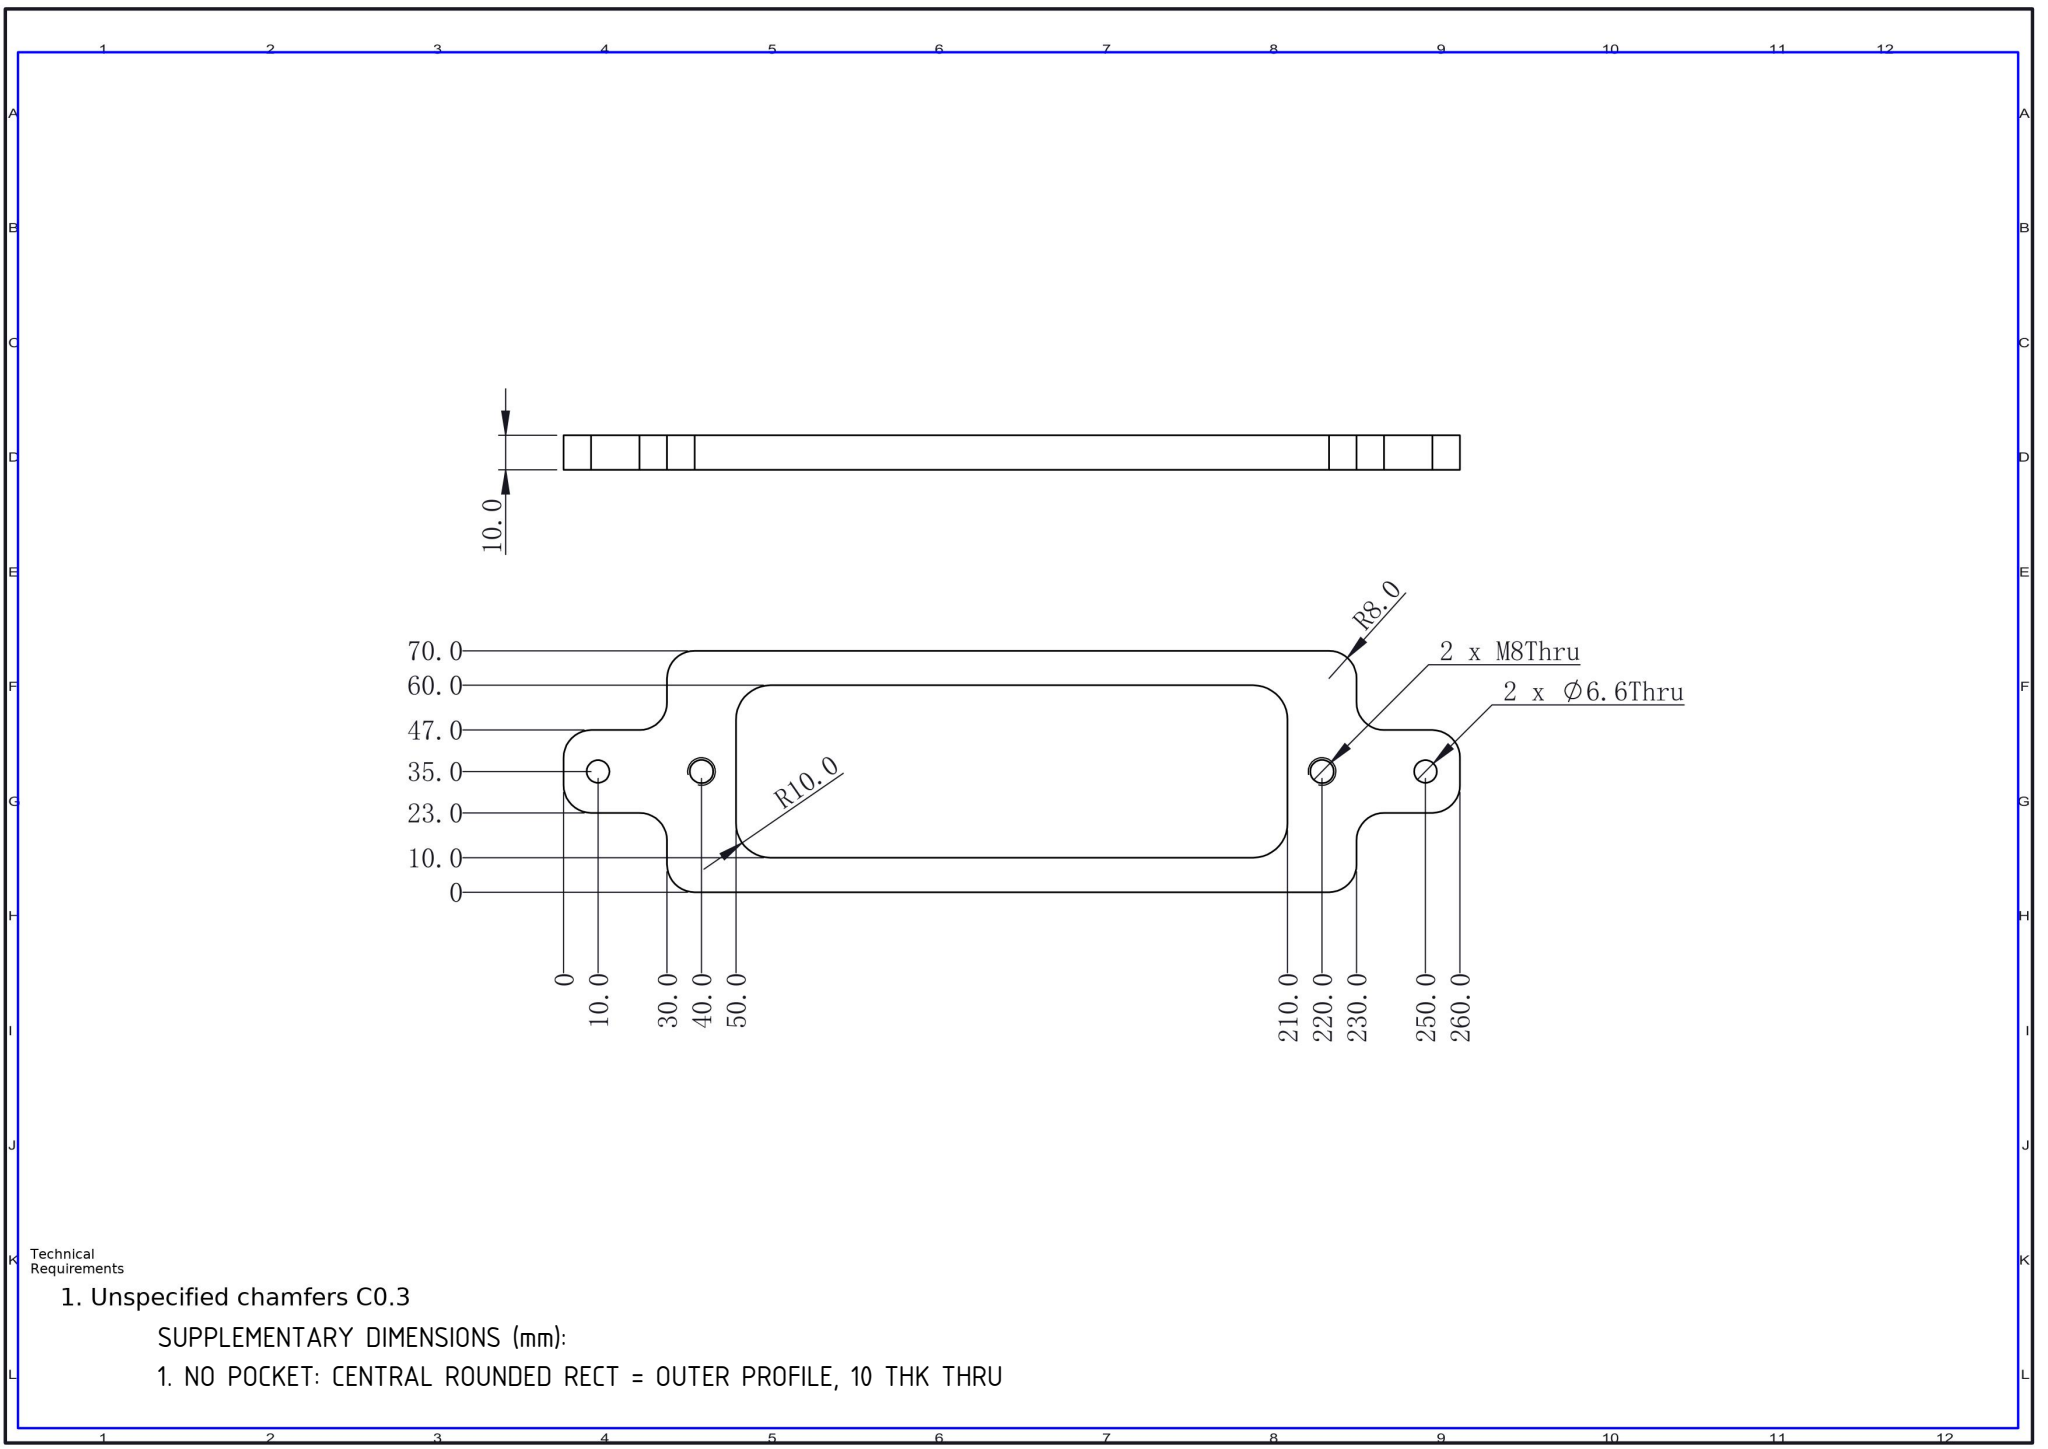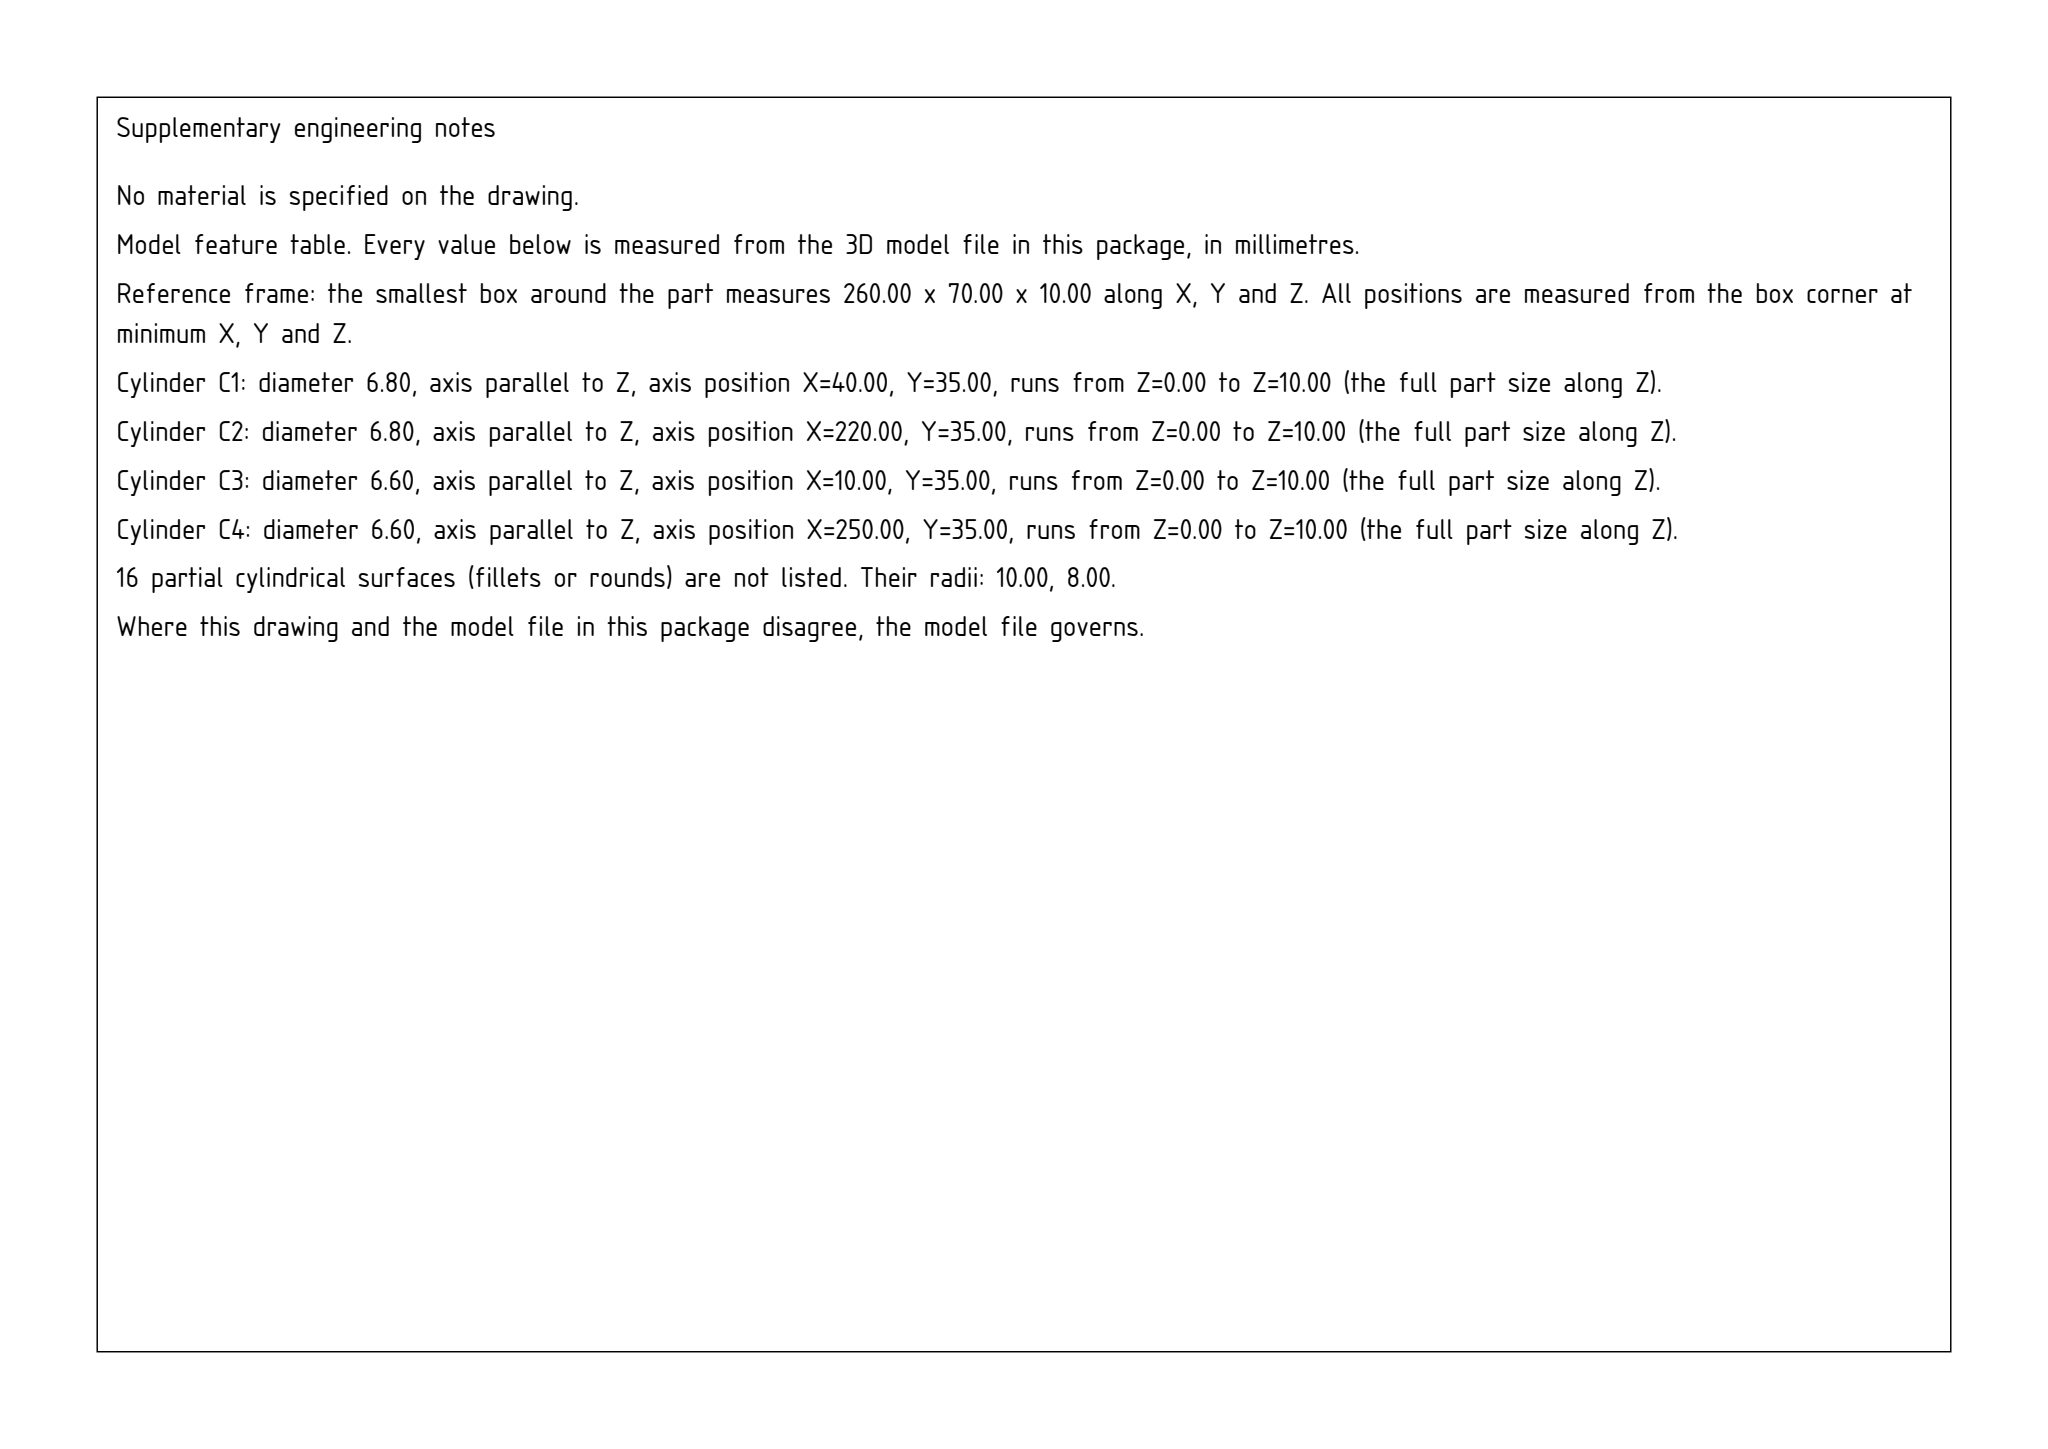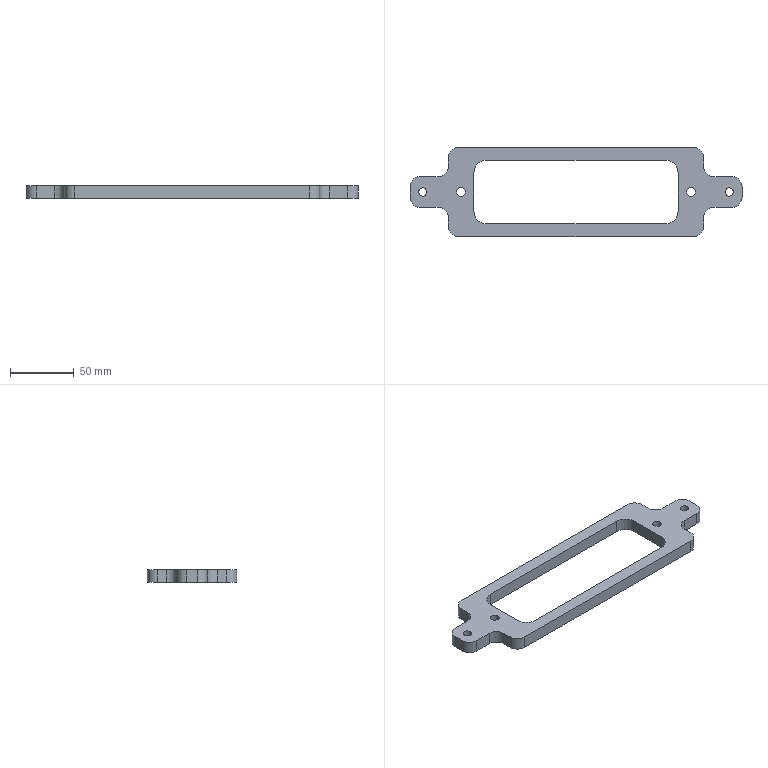Part | SolidWorks | mm | 1 solid | 42 faces | box 260 x 70 x 10 mm | volume 73298 mm3 | cylinder 24 | plane 18 | commonest cylinder face diameters 16 x12 6.8 x4 6.6 x4 20 x4
build123d program:
from build123d import *

# Parameters (mm, degrees)
SKETCH1_W            = 260
SKETCH1_H            = 70
BOSS_EXTRUDE1_DEPTH  = 10
SKETCH2_W            = 30
SKETCH2_H            = 23
CUT_EXTRUDE1_DEPTH   = 136
FILLET1_R            = 8
M6_CLEARANCE_HOLE1_D = 6.6
M8_TAPPED_HOLE1_D    = 6.8


with BuildPart() as part:
    # Sketch1 → Boss-Extrude1 (new body)
    with BuildSketch(Plane.XY):
        Rectangle(SKETCH1_W, SKETCH1_H)
        with BuildLine():
            Line((-70, 25), (70, 25))
            ThreePointArc((70, 25), (77.071, 22.071), (80, 15))
            Line((80, 15), (80, -15))
            ThreePointArc((80, -15), (77.071, -22.071), (70, -25))
            Line((70, -25), (-70, -25))
            ThreePointArc((-70, -25), (-77.071, -22.071), (-80, -15))
            Line((-80, -15), (-80, 15))
            ThreePointArc((-80, 15), (-77.071, 22.071), (-70, 25))
        make_face(mode=Mode.SUBTRACT)
    extrude(amount=BOSS_EXTRUDE1_DEPTH)

    # Sketch2 → Cut-Extrude1 (cut, through all)
    with BuildSketch(Plane.XY.offset(10)):
        with Locations((-115, 23.5)):
            Rectangle(SKETCH2_W, SKETCH2_H)
        with Locations((-115, -23.5)):
            Rectangle(SKETCH2_W, SKETCH2_H)
        with Locations((115, -23.5)):
            Rectangle(SKETCH2_W, SKETCH2_H)
        with Locations((115, 23.5)):
            Rectangle(SKETCH2_W, SKETCH2_H)
    extrude(amount=-CUT_EXTRUDE1_DEPTH, mode=Mode.SUBTRACT)

    # Fillet1
    fillet1_edges = [part.edges().sort_by_distance(p)[0] for p in [
        (130, 12, 5),
        (100, 12, 5),
        (100, 35, 5),
        (130, -12, 5),
        (100, -35, 5),
        (100, -12, 5),
        (-130, -12, 5),
        (-100, -12, 5),
        (-100, -35, 5),
        (-130, 12, 5),
        (-100, 35, 5),
        (-100, 12, 5),
    ]]
    fillet(fillet1_edges, radius=FILLET1_R)

    # M6 Clearance Hole1 (through all)
    with Locations(Plane(origin=(0, 0, 0), x_dir=(-1, 0, 0), z_dir=(0, 0, -1))):
        with Locations((-120, 0), (120, 0)):
            Hole(M6_CLEARANCE_HOLE1_D / 2)

    # M8 Tapped Hole1 (through all)
    with Locations(Plane(origin=(0, 0, 0), x_dir=(-1, 0, 0), z_dir=(0, 0, -1))):
        with Locations((-90, 0), (90, 0)):
            Hole(M8_TAPPED_HOLE1_D / 2)


with BuildPart() as part_1:
    # Body-Move_Copy1: moved
    add(part.part.moved(Location((0, 0, -10))))


solid = part_1.part